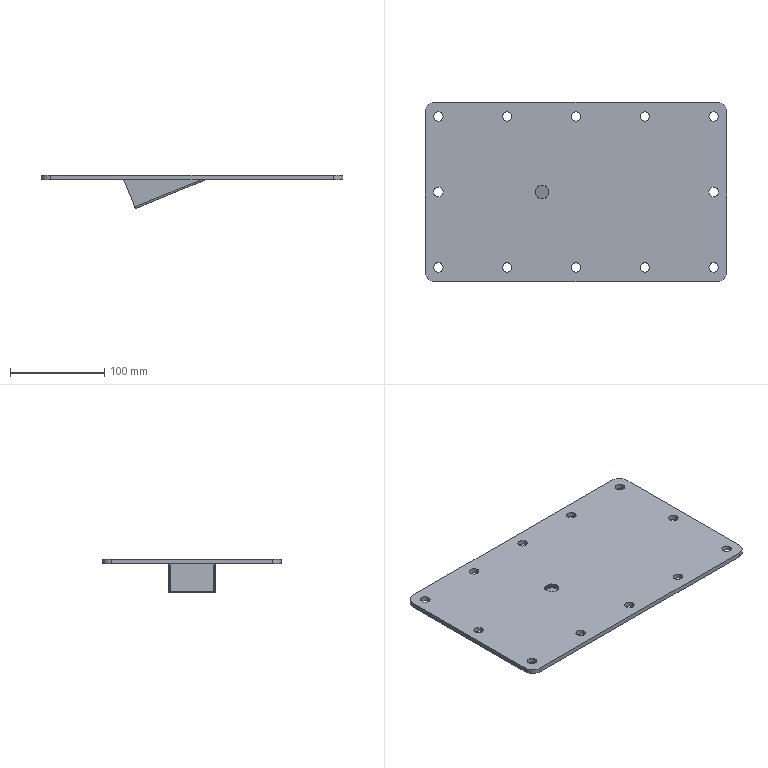Component | NX | T5_COVER_PLATE | 2 solids | 39 faces | volume 304263 mm3 | cylinder 22 | plane 15 | spline 2 | commonest cylinder face diameters 10 x12 20 x4 4 x2 2 x2 14.5 x1 16 x1